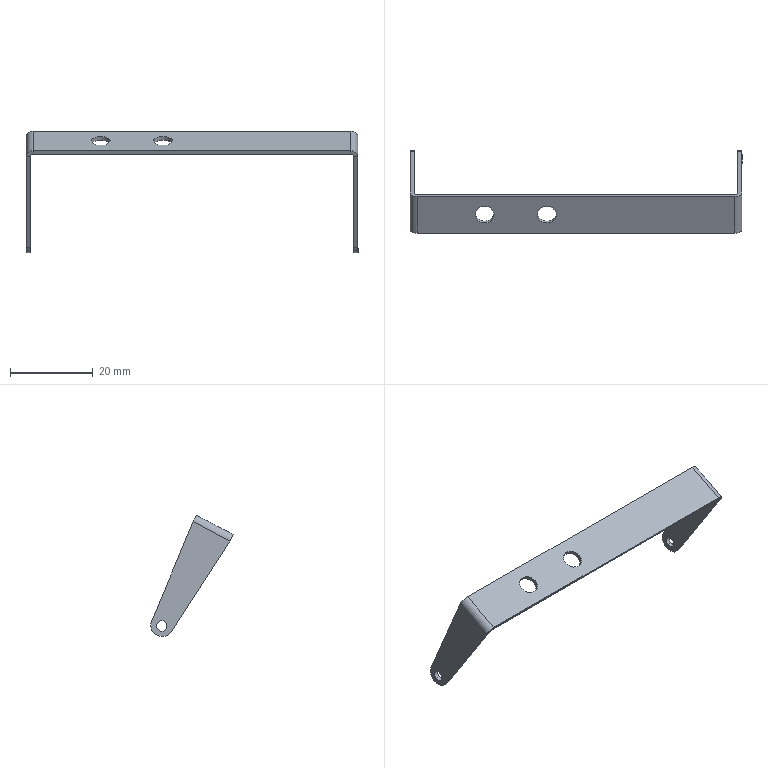Component | SolidWorks | ToolHolderAssembly-1_ToolHolder-1 | 1 solid | 34 faces | box 80 x 19.87 x 29.24 mm | volume 1182 mm3 | plane 18 | cylinder 16 | commonest cylinder face diameters 4.5 x4 2.5 x4 5.2 x4 3.473 x2 1.473 x2
STEP:
#1=COLOUR_RGB('',0.7922,0.8196,0.9333);
#2=FILL_AREA_STYLE_COLOUR('',#1);
#3=FILL_AREA_STYLE('',(#2));
#4=SURFACE_STYLE_FILL_AREA(#3);
#5=SURFACE_SIDE_STYLE('',(#4));
#6=SURFACE_STYLE_USAGE(.BOTH.,#5);
#7=PRESENTATION_STYLE_ASSIGNMENT((#6));
#8=CARTESIAN_POINT('',(-6.282,-0.2465,6.428));
#9=VERTEX_POINT('',#8);
#10=CARTESIAN_POINT('',(-6.105,-0.2465,6.428));
#11=VERTEX_POINT('',#10);
#12=CARTESIAN_POINT('',(-6.194,-0.2465,6.428));
#13=DIRECTION('',(-0.,-0.4648,0.8854));
#14=DIRECTION('',(1.,-0.,0.));
#15=AXIS2_PLACEMENT_3D('',#12,#13,#14);
#16=CIRCLE('',#15,0.08858);
#17=EDGE_CURVE('',#9,#11,#16,.T.);
#18=ORIENTED_EDGE('',*,*,#17,.F.);
#19=CARTESIAN_POINT('',(-6.282,-0.2648,6.463));
#20=VERTEX_POINT('',#19);
#21=CARTESIAN_POINT('',(-6.282,-0.2648,6.463));
#22=DIRECTION('',(-0.,-0.4648,0.8854));
#23=VECTOR('',#22,39.37);
#24=LINE('',#21,#23);
#25=EDGE_CURVE('',#9,#20,#24,.T.);
#26=ORIENTED_EDGE('',*,*,#25,.T.);
#27=CARTESIAN_POINT('',(-6.105,-0.2648,6.463));
#28=VERTEX_POINT('',#27);
#29=CARTESIAN_POINT('',(-6.194,-0.2648,6.463));
#30=DIRECTION('',(-0.,-0.4648,0.8854));
#31=DIRECTION('',(1.,-0.,0.));
#32=AXIS2_PLACEMENT_3D('',#29,#30,#31);
#33=CIRCLE('',#32,0.08858);
#34=EDGE_CURVE('',#20,#28,#33,.T.);
#35=ORIENTED_EDGE('',*,*,#34,.T.);
#36=CARTESIAN_POINT('',(-6.105,-0.2648,6.463));
#37=DIRECTION('',(-0.,-0.4648,0.8854));
#38=VECTOR('',#37,39.37);
#39=LINE('',#36,#38);
#40=EDGE_CURVE('',#11,#28,#39,.T.);
#41=ORIENTED_EDGE('',*,*,#40,.F.);
#42=EDGE_LOOP('',(#18,#26,#35,#41));
#43=FACE_OUTER_BOUND('',#42,.T.);
#44=CARTESIAN_POINT('',(-6.194,-0.2648,6.463));
#45=DIRECTION('',(-0.,-0.4648,0.8854));
#46=DIRECTION('',(1.,-0.,0.));
#47=AXIS2_PLACEMENT_3D('',#44,#45,#46);
#48=CYLINDRICAL_SURFACE('',#47,0.08858);
#49=ADVANCED_FACE('',(#43),#48,.F.);
#50=CARTESIAN_POINT('',(-6.873,-0.2465,6.428));
#51=VERTEX_POINT('',#50);
#52=CARTESIAN_POINT('',(-6.696,-0.2465,6.428));
#53=VERTEX_POINT('',#52);
#54=CARTESIAN_POINT('',(-6.784,-0.2465,6.428));
#55=DIRECTION('',(-0.,-0.4648,0.8854));
#56=DIRECTION('',(1.,-0.,0.));
#57=AXIS2_PLACEMENT_3D('',#54,#55,#56);
#58=CIRCLE('',#57,0.08858);
#59=EDGE_CURVE('',#51,#53,#58,.T.);
#60=ORIENTED_EDGE('',*,*,#59,.F.);
#61=CARTESIAN_POINT('',(-6.873,-0.2648,6.463));
#62=VERTEX_POINT('',#61);
#63=CARTESIAN_POINT('',(-6.873,-0.2648,6.463));
#64=DIRECTION('',(-0.,-0.4648,0.8854));
#65=VECTOR('',#64,39.37);
#66=LINE('',#63,#65);
#67=EDGE_CURVE('',#51,#62,#66,.T.);
#68=ORIENTED_EDGE('',*,*,#67,.T.);
#69=CARTESIAN_POINT('',(-6.696,-0.2648,6.463));
#70=VERTEX_POINT('',#69);
#71=CARTESIAN_POINT('',(-6.784,-0.2648,6.463));
#72=DIRECTION('',(-0.,-0.4648,0.8854));
#73=DIRECTION('',(1.,-0.,0.));
#74=AXIS2_PLACEMENT_3D('',#71,#72,#73);
#75=CIRCLE('',#74,0.08858);
#76=EDGE_CURVE('',#62,#70,#75,.T.);
#77=ORIENTED_EDGE('',*,*,#76,.T.);
#78=CARTESIAN_POINT('',(-6.696,-0.2648,6.463));
#79=DIRECTION('',(-0.,-0.4648,0.8854));
#80=VECTOR('',#79,39.37);
#81=LINE('',#78,#80);
#82=EDGE_CURVE('',#53,#70,#81,.T.);
#83=ORIENTED_EDGE('',*,*,#82,.F.);
#84=EDGE_LOOP('',(#60,#68,#77,#83));
#85=FACE_OUTER_BOUND('',#84,.T.);
#86=CARTESIAN_POINT('',(-6.784,-0.2648,6.463));
#87=DIRECTION('',(-0.,-0.4648,0.8854));
#88=DIRECTION('',(1.,-0.,0.));
#89=AXIS2_PLACEMENT_3D('',#86,#87,#88);
#90=CYLINDRICAL_SURFACE('',#89,0.08858);
#91=ADVANCED_FACE('',(#85),#90,.F.);
#92=CARTESIAN_POINT('',(-4.383,0.2613,5.461));
#93=VERTEX_POINT('',#92);
#94=CARTESIAN_POINT('',(-4.383,0.2155,5.548));
#95=VERTEX_POINT('',#94);
#96=CARTESIAN_POINT('',(-4.383,0.2384,5.504));
#97=DIRECTION('',(-1.,0.,-0.));
#98=DIRECTION('',(-0.,-0.4648,0.8854));
#99=AXIS2_PLACEMENT_3D('',#96,#97,#98);
#100=CIRCLE('',#99,0.04921);
#101=EDGE_CURVE('',#93,#95,#100,.T.);
#102=ORIENTED_EDGE('',*,*,#101,.T.);
#103=CARTESIAN_POINT('',(-4.343,0.2155,5.548));
#104=VERTEX_POINT('',#103);
#105=CARTESIAN_POINT('',(-7.493,0.2155,5.548));
#106=DIRECTION('',(1.,-0.,0.));
#107=VECTOR('',#106,39.37);
#108=LINE('',#105,#107);
#109=EDGE_CURVE('',#95,#104,#108,.T.);
#110=ORIENTED_EDGE('',*,*,#109,.T.);
#111=CARTESIAN_POINT('',(-4.343,0.2613,5.461));
#112=VERTEX_POINT('',#111);
#113=CARTESIAN_POINT('',(-4.343,0.2384,5.504));
#114=DIRECTION('',(1.,-0.,0.));
#115=DIRECTION('',(0.,0.4648,-0.8854));
#116=AXIS2_PLACEMENT_3D('',#113,#114,#115);
#117=CIRCLE('',#116,0.04921);
#118=EDGE_CURVE('',#104,#112,#117,.T.);
#119=ORIENTED_EDGE('',*,*,#118,.T.);
#120=CARTESIAN_POINT('',(-7.493,0.2613,5.461));
#121=DIRECTION('',(1.,-0.,0.));
#122=VECTOR('',#121,39.37);
#123=LINE('',#120,#122);
#124=EDGE_CURVE('',#93,#112,#123,.T.);
#125=ORIENTED_EDGE('',*,*,#124,.F.);
#126=EDGE_LOOP('',(#102,#110,#119,#125));
#127=FACE_OUTER_BOUND('',#126,.T.);
#128=CARTESIAN_POINT('',(-7.493,0.2384,5.504));
#129=DIRECTION('',(1.,-0.,0.));
#130=DIRECTION('',(0.,0.4648,-0.8854));
#131=AXIS2_PLACEMENT_3D('',#128,#129,#130);
#132=CYLINDRICAL_SURFACE('',#131,0.04921);
#133=ADVANCED_FACE('',(#127),#132,.F.);
#134=CARTESIAN_POINT('',(-7.493,0.2155,5.548));
#135=VERTEX_POINT('',#134);
#136=CARTESIAN_POINT('',(-7.493,0.2613,5.461));
#137=VERTEX_POINT('',#136);
#138=CARTESIAN_POINT('',(-7.493,0.2384,5.504));
#139=DIRECTION('',(1.,-0.,0.));
#140=DIRECTION('',(0.,0.4648,-0.8854));
#141=AXIS2_PLACEMENT_3D('',#138,#139,#140);
#142=CIRCLE('',#141,0.04921);
#143=EDGE_CURVE('',#135,#137,#142,.T.);
#144=ORIENTED_EDGE('',*,*,#143,.F.);
#145=CARTESIAN_POINT('',(-7.453,0.2155,5.548));
#146=VERTEX_POINT('',#145);
#147=CARTESIAN_POINT('',(-7.493,0.2155,5.548));
#148=DIRECTION('',(1.,-0.,0.));
#149=VECTOR('',#148,39.37);
#150=LINE('',#147,#149);
#151=EDGE_CURVE('',#135,#146,#150,.T.);
#152=ORIENTED_EDGE('',*,*,#151,.T.);
#153=CARTESIAN_POINT('',(-7.453,0.2613,5.461));
#154=VERTEX_POINT('',#153);
#155=CARTESIAN_POINT('',(-7.453,0.2384,5.504));
#156=DIRECTION('',(1.,-0.,0.));
#157=DIRECTION('',(0.,0.4648,-0.8854));
#158=AXIS2_PLACEMENT_3D('',#155,#156,#157);
#159=CIRCLE('',#158,0.04921);
#160=EDGE_CURVE('',#146,#154,#159,.T.);
#161=ORIENTED_EDGE('',*,*,#160,.T.);
#162=CARTESIAN_POINT('',(-7.493,0.2613,5.461));
#163=DIRECTION('',(1.,-0.,0.));
#164=VECTOR('',#163,39.37);
#165=LINE('',#162,#164);
#166=EDGE_CURVE('',#137,#154,#165,.T.);
#167=ORIENTED_EDGE('',*,*,#166,.F.);
#168=EDGE_LOOP('',(#144,#152,#161,#167));
#169=FACE_OUTER_BOUND('',#168,.T.);
#170=CARTESIAN_POINT('',(-7.493,0.2384,5.504));
#171=DIRECTION('',(1.,-0.,0.));
#172=DIRECTION('',(0.,0.4648,-0.8854));
#173=AXIS2_PLACEMENT_3D('',#170,#171,#172);
#174=CYLINDRICAL_SURFACE('',#173,0.04921);
#175=ADVANCED_FACE('',(#169),#174,.F.);
#176=CARTESIAN_POINT('',(-6.194,-0.2648,6.463));
#177=DIRECTION('',(-0.,-0.4648,0.8854));
#178=DIRECTION('',(1.,-0.,0.));
#179=AXIS2_PLACEMENT_3D('',#176,#177,#178);
#180=CIRCLE('',#179,0.08858);
#181=EDGE_CURVE('',#28,#20,#180,.T.);
#182=ORIENTED_EDGE('',*,*,#181,.F.);
#183=ORIENTED_EDGE('',*,*,#34,.F.);
#184=EDGE_LOOP('',(#182,#183));
#185=FACE_BOUND('',#184,.T.);
#186=CARTESIAN_POINT('',(-6.784,-0.2648,6.463));
#187=DIRECTION('',(-0.,-0.4648,0.8854));
#188=DIRECTION('',(1.,-0.,0.));
#189=AXIS2_PLACEMENT_3D('',#186,#187,#188);
#190=CIRCLE('',#189,0.08858);
#191=EDGE_CURVE('',#70,#62,#190,.T.);
#192=ORIENTED_EDGE('',*,*,#191,.F.);
#193=ORIENTED_EDGE('',*,*,#76,.F.);
#194=EDGE_LOOP('',(#192,#193));
#195=FACE_BOUND('',#194,.T.);
#196=CARTESIAN_POINT('',(-7.424,-0.09053,6.554));
#197=VERTEX_POINT('',#196);
#198=CARTESIAN_POINT('',(-4.412,-0.09053,6.554));
#199=VERTEX_POINT('',#198);
#200=CARTESIAN_POINT('',(-4.343,-0.09053,6.554));
#201=DIRECTION('',(1.,-0.,0.));
#202=VECTOR('',#201,39.37);
#203=LINE('',#200,#202);
#204=EDGE_CURVE('',#197,#199,#203,.T.);
#205=ORIENTED_EDGE('',*,*,#204,.F.);
#206=CARTESIAN_POINT('',(-7.424,-0.4391,6.371));
#207=VERTEX_POINT('',#206);
#208=CARTESIAN_POINT('',(-7.424,-0.09053,6.554));
#209=DIRECTION('',(0.,-0.8854,-0.4648));
#210=VECTOR('',#209,39.37);
#211=LINE('',#208,#210);
#212=EDGE_CURVE('',#197,#207,#211,.T.);
#213=ORIENTED_EDGE('',*,*,#212,.T.);
#214=CARTESIAN_POINT('',(-4.412,-0.4391,6.371));
#215=VERTEX_POINT('',#214);
#216=CARTESIAN_POINT('',(-4.343,-0.4391,6.371));
#217=DIRECTION('',(-1.,0.,-0.));
#218=VECTOR('',#217,39.37);
#219=LINE('',#216,#218);
#220=EDGE_CURVE('',#215,#207,#219,.T.);
#221=ORIENTED_EDGE('',*,*,#220,.F.);
#222=CARTESIAN_POINT('',(-4.412,-0.4391,6.371));
#223=DIRECTION('',(-0.,0.8854,0.4648));
#224=VECTOR('',#223,39.37);
#225=LINE('',#222,#224);
#226=EDGE_CURVE('',#215,#199,#225,.T.);
#227=ORIENTED_EDGE('',*,*,#226,.T.);
#228=EDGE_LOOP('',(#205,#213,#221,#227));
#229=FACE_OUTER_BOUND('',#228,.T.);
#230=CARTESIAN_POINT('',(-5.918,-0.2648,6.463));
#231=DIRECTION('',(-0.,-0.4648,0.8854));
#232=DIRECTION('',(1.,-0.,0.));
#233=AXIS2_PLACEMENT_3D('',#230,#231,#232);
#234=PLANE('',#233);
#235=ADVANCED_FACE('',(#185,#195,#229),#234,.T.);
#236=CARTESIAN_POINT('',(-6.194,-0.2465,6.428));
#237=DIRECTION('',(-0.,-0.4648,0.8854));
#238=DIRECTION('',(1.,-0.,0.));
#239=AXIS2_PLACEMENT_3D('',#236,#237,#238);
#240=CIRCLE('',#239,0.08858);
#241=EDGE_CURVE('',#11,#9,#240,.T.);
#242=ORIENTED_EDGE('',*,*,#241,.T.);
#243=ORIENTED_EDGE('',*,*,#17,.T.);
#244=EDGE_LOOP('',(#242,#243));
#245=FACE_BOUND('',#244,.T.);
#246=CARTESIAN_POINT('',(-6.784,-0.2465,6.428));
#247=DIRECTION('',(-0.,-0.4648,0.8854));
#248=DIRECTION('',(1.,-0.,0.));
#249=AXIS2_PLACEMENT_3D('',#246,#247,#248);
#250=CIRCLE('',#249,0.08858);
#251=EDGE_CURVE('',#53,#51,#250,.T.);
#252=ORIENTED_EDGE('',*,*,#251,.T.);
#253=ORIENTED_EDGE('',*,*,#59,.T.);
#254=EDGE_LOOP('',(#252,#253));
#255=FACE_BOUND('',#254,.T.);
#256=CARTESIAN_POINT('',(-7.424,-0.07223,6.52));
#257=VERTEX_POINT('',#256);
#258=CARTESIAN_POINT('',(-7.424,-0.4208,6.337));
#259=VERTEX_POINT('',#258);
#260=CARTESIAN_POINT('',(-7.424,-0.07223,6.52));
#261=DIRECTION('',(0.,-0.8854,-0.4648));
#262=VECTOR('',#261,39.37);
#263=LINE('',#260,#262);
#264=EDGE_CURVE('',#257,#259,#263,.T.);
#265=ORIENTED_EDGE('',*,*,#264,.F.);
#266=CARTESIAN_POINT('',(-4.412,-0.07223,6.52));
#267=VERTEX_POINT('',#266);
#268=CARTESIAN_POINT('',(-4.343,-0.07223,6.52));
#269=DIRECTION('',(1.,-0.,0.));
#270=VECTOR('',#269,39.37);
#271=LINE('',#268,#270);
#272=EDGE_CURVE('',#257,#267,#271,.T.);
#273=ORIENTED_EDGE('',*,*,#272,.T.);
#274=CARTESIAN_POINT('',(-4.412,-0.4208,6.337));
#275=VERTEX_POINT('',#274);
#276=CARTESIAN_POINT('',(-4.412,-0.4208,6.337));
#277=DIRECTION('',(-0.,0.8854,0.4648));
#278=VECTOR('',#277,39.37);
#279=LINE('',#276,#278);
#280=EDGE_CURVE('',#275,#267,#279,.T.);
#281=ORIENTED_EDGE('',*,*,#280,.F.);
#282=CARTESIAN_POINT('',(-4.343,-0.4208,6.337));
#283=DIRECTION('',(-1.,0.,-0.));
#284=VECTOR('',#283,39.37);
#285=LINE('',#282,#284);
#286=EDGE_CURVE('',#275,#259,#285,.T.);
#287=ORIENTED_EDGE('',*,*,#286,.T.);
#288=EDGE_LOOP('',(#265,#273,#281,#287));
#289=FACE_OUTER_BOUND('',#288,.T.);
#290=CARTESIAN_POINT('',(-5.918,-0.2465,6.428));
#291=DIRECTION('',(-0.,-0.4648,0.8854));
#292=DIRECTION('',(1.,-0.,0.));
#293=AXIS2_PLACEMENT_3D('',#290,#291,#292);
#294=PLANE('',#293);
#295=ADVANCED_FACE('',(#245,#255,#289),#294,.F.);
#296=ORIENTED_EDGE('',*,*,#272,.F.);
#297=CARTESIAN_POINT('',(-7.424,-0.07223,6.52));
#298=DIRECTION('',(-0.,-0.4648,0.8854));
#299=VECTOR('',#298,39.37);
#300=LINE('',#297,#299);
#301=EDGE_CURVE('',#257,#197,#300,.T.);
#302=ORIENTED_EDGE('',*,*,#301,.T.);
#303=ORIENTED_EDGE('',*,*,#204,.T.);
#304=CARTESIAN_POINT('',(-4.412,-0.07223,6.52));
#305=DIRECTION('',(-0.,-0.4648,0.8854));
#306=VECTOR('',#305,39.37);
#307=LINE('',#304,#306);
#308=EDGE_CURVE('',#267,#199,#307,.T.);
#309=ORIENTED_EDGE('',*,*,#308,.F.);
#310=EDGE_LOOP('',(#296,#302,#303,#309));
#311=FACE_OUTER_BOUND('',#310,.T.);
#312=CARTESIAN_POINT('',(-4.343,-0.09053,6.554));
#313=DIRECTION('',(-0.,0.8854,0.4648));
#314=DIRECTION('',(0.,0.4648,-0.8854));
#315=AXIS2_PLACEMENT_3D('',#312,#313,#314);
#316=PLANE('',#315);
#317=ADVANCED_FACE('',(#311),#316,.T.);
#318=CARTESIAN_POINT('',(-7.424,-0.4208,6.337));
#319=DIRECTION('',(-0.,-0.4648,0.8854));
#320=VECTOR('',#319,39.37);
#321=LINE('',#318,#320);
#322=EDGE_CURVE('',#259,#207,#321,.T.);
#323=ORIENTED_EDGE('',*,*,#322,.F.);
#324=ORIENTED_EDGE('',*,*,#286,.F.);
#325=CARTESIAN_POINT('',(-4.412,-0.4208,6.337));
#326=DIRECTION('',(-0.,-0.4648,0.8854));
#327=VECTOR('',#326,39.37);
#328=LINE('',#325,#327);
#329=EDGE_CURVE('',#275,#215,#328,.T.);
#330=ORIENTED_EDGE('',*,*,#329,.T.);
#331=ORIENTED_EDGE('',*,*,#220,.T.);
#332=EDGE_LOOP('',(#323,#324,#330,#331));
#333=FACE_OUTER_BOUND('',#332,.T.);
#334=CARTESIAN_POINT('',(-4.343,-0.4391,6.371));
#335=DIRECTION('',(0.,-0.8854,-0.4648));
#336=DIRECTION('',(-0.,-0.4648,0.8854));
#337=AXIS2_PLACEMENT_3D('',#334,#335,#336);
#338=PLANE('',#337);
#339=ADVANCED_FACE('',(#333),#338,.T.);
#340=CARTESIAN_POINT('',(-4.383,-0.05875,6.494));
#341=VERTEX_POINT('',#340);
#342=CARTESIAN_POINT('',(-4.343,-0.05875,6.494));
#343=VERTEX_POINT('',#342);
#344=CARTESIAN_POINT('',(-4.343,-0.05875,6.494));
#345=DIRECTION('',(1.,-0.,0.));
#346=VECTOR('',#345,39.37);
#347=LINE('',#344,#346);
#348=EDGE_CURVE('',#341,#343,#347,.T.);
#349=ORIENTED_EDGE('',*,*,#348,.F.);
#350=CARTESIAN_POINT('',(-4.412,-0.05875,6.494));
#351=DIRECTION('',(-0.,0.8854,0.4648));
#352=DIRECTION('',(-0.,-0.4648,0.8854));
#353=AXIS2_PLACEMENT_3D('',#350,#351,#352);
#354=CIRCLE('',#353,0.029);
#355=EDGE_CURVE('',#267,#341,#354,.T.);
#356=ORIENTED_EDGE('',*,*,#355,.F.);
#357=ORIENTED_EDGE('',*,*,#308,.T.);
#358=CARTESIAN_POINT('',(-4.412,-0.05875,6.494));
#359=DIRECTION('',(-0.,0.8854,0.4648));
#360=DIRECTION('',(-0.,-0.4648,0.8854));
#361=AXIS2_PLACEMENT_3D('',#358,#359,#360);
#362=CIRCLE('',#361,0.06837);
#363=EDGE_CURVE('',#199,#343,#362,.T.);
#364=ORIENTED_EDGE('',*,*,#363,.T.);
#365=EDGE_LOOP('',(#349,#356,#357,#364));
#366=FACE_OUTER_BOUND('',#365,.T.);
#367=CARTESIAN_POINT('',(-4.412,-0.05875,6.494));
#368=DIRECTION('',(-0.,0.8854,0.4648));
#369=DIRECTION('',(0.,0.4648,-0.8854));
#370=AXIS2_PLACEMENT_3D('',#367,#368,#369);
#371=PLANE('',#370);
#372=ADVANCED_FACE('',(#366),#371,.T.);
#373=CARTESIAN_POINT('',(-4.383,-0.4073,6.311));
#374=VERTEX_POINT('',#373);
#375=CARTESIAN_POINT('',(-4.412,-0.4073,6.311));
#376=DIRECTION('',(0.,-0.8854,-0.4648));
#377=DIRECTION('',(-0.,-0.4648,0.8854));
#378=AXIS2_PLACEMENT_3D('',#375,#376,#377);
#379=CIRCLE('',#378,0.029);
#380=EDGE_CURVE('',#374,#275,#379,.T.);
#381=ORIENTED_EDGE('',*,*,#380,.F.);
#382=CARTESIAN_POINT('',(-4.343,-0.4073,6.311));
#383=VERTEX_POINT('',#382);
#384=CARTESIAN_POINT('',(-4.383,-0.4073,6.311));
#385=DIRECTION('',(1.,-0.,0.));
#386=VECTOR('',#385,39.37);
#387=LINE('',#384,#386);
#388=EDGE_CURVE('',#374,#383,#387,.T.);
#389=ORIENTED_EDGE('',*,*,#388,.T.);
#390=CARTESIAN_POINT('',(-4.412,-0.4073,6.311));
#391=DIRECTION('',(0.,-0.8854,-0.4648));
#392=DIRECTION('',(-0.,-0.4648,0.8854));
#393=AXIS2_PLACEMENT_3D('',#390,#391,#392);
#394=CIRCLE('',#393,0.06837);
#395=EDGE_CURVE('',#383,#215,#394,.T.);
#396=ORIENTED_EDGE('',*,*,#395,.T.);
#397=ORIENTED_EDGE('',*,*,#329,.F.);
#398=EDGE_LOOP('',(#381,#389,#396,#397));
#399=FACE_OUTER_BOUND('',#398,.T.);
#400=CARTESIAN_POINT('',(-4.412,-0.4073,6.311));
#401=DIRECTION('',(-0.,0.8854,0.4648));
#402=DIRECTION('',(0.,0.4648,-0.8854));
#403=AXIS2_PLACEMENT_3D('',#400,#401,#402);
#404=PLANE('',#403);
#405=ADVANCED_FACE('',(#399),#404,.F.);
#406=ORIENTED_EDGE('',*,*,#226,.F.);
#407=ORIENTED_EDGE('',*,*,#395,.F.);
#408=CARTESIAN_POINT('',(-4.343,-0.05875,6.494));
#409=DIRECTION('',(-0.,0.8854,0.4648));
#410=VECTOR('',#409,39.37);
#411=LINE('',#408,#410);
#412=EDGE_CURVE('',#383,#343,#411,.T.);
#413=ORIENTED_EDGE('',*,*,#412,.T.);
#414=ORIENTED_EDGE('',*,*,#363,.F.);
#415=EDGE_LOOP('',(#406,#407,#413,#414));
#416=FACE_OUTER_BOUND('',#415,.T.);
#417=CARTESIAN_POINT('',(-4.412,-0.4073,6.311));
#418=DIRECTION('',(0.,-0.8854,-0.4648));
#419=DIRECTION('',(1.,-0.,0.));
#420=AXIS2_PLACEMENT_3D('',#417,#418,#419);
#421=CYLINDRICAL_SURFACE('',#420,0.06837);
#422=ADVANCED_FACE('',(#416),#421,.T.);
#423=ORIENTED_EDGE('',*,*,#280,.T.);
#424=ORIENTED_EDGE('',*,*,#355,.T.);
#425=CARTESIAN_POINT('',(-4.383,-0.05875,6.494));
#426=DIRECTION('',(0.,-0.8854,-0.4648));
#427=VECTOR('',#426,39.37);
#428=LINE('',#425,#427);
#429=EDGE_CURVE('',#341,#374,#428,.T.);
#430=ORIENTED_EDGE('',*,*,#429,.T.);
#431=ORIENTED_EDGE('',*,*,#380,.T.);
#432=EDGE_LOOP('',(#423,#424,#430,#431));
#433=FACE_OUTER_BOUND('',#432,.T.);
#434=CARTESIAN_POINT('',(-4.412,-0.4073,6.311));
#435=DIRECTION('',(0.,-0.8854,-0.4648));
#436=DIRECTION('',(1.,-0.,0.));
#437=AXIS2_PLACEMENT_3D('',#434,#435,#436);
#438=CYLINDRICAL_SURFACE('',#437,0.029);
#439=ADVANCED_FACE('',(#433),#438,.F.);
#440=CARTESIAN_POINT('',(-4.343,0.2384,5.504));
#441=DIRECTION('',(1.,-0.,0.));
#442=DIRECTION('',(0.,0.4648,-0.8854));
#443=AXIS2_PLACEMENT_3D('',#440,#441,#442);
#444=CIRCLE('',#443,0.04921);
#445=EDGE_CURVE('',#112,#104,#444,.T.);
#446=ORIENTED_EDGE('',*,*,#445,.F.);
#447=ORIENTED_EDGE('',*,*,#118,.F.);
#448=EDGE_LOOP('',(#446,#447));
#449=FACE_BOUND('',#448,.T.);
#450=CARTESIAN_POINT('',(-4.343,0.28,5.415));
#451=VERTEX_POINT('',#450);
#452=CARTESIAN_POINT('',(-4.343,0.2883,5.419));
#453=VERTEX_POINT('',#452);
#454=CARTESIAN_POINT('',(-4.343,0.2842,5.417));
#455=DIRECTION('',(-0.,0.8854,0.4648));
#456=VECTOR('',#455,39.37);
#457=LINE('',#454,#456);
#458=EDGE_CURVE('',#451,#453,#457,.T.);
#459=ORIENTED_EDGE('',*,*,#458,.T.);
#460=CARTESIAN_POINT('',(-4.343,0.3352,5.549));
#461=VERTEX_POINT('',#460);
#462=CARTESIAN_POINT('',(-4.343,0.2408,5.51));
#463=DIRECTION('',(1.,-0.,0.));
#464=DIRECTION('',(-0.,-0.4648,0.8854));
#465=AXIS2_PLACEMENT_3D('',#462,#463,#464);
#466=CIRCLE('',#465,0.1024);
#467=EDGE_CURVE('',#453,#461,#466,.T.);
#468=ORIENTED_EDGE('',*,*,#467,.T.);
#469=CARTESIAN_POINT('',(-4.343,-0.05875,6.494));
#470=DIRECTION('',(0.,0.385,-0.9229));
#471=VECTOR('',#470,39.37);
#472=LINE('',#469,#471);
#473=EDGE_CURVE('',#343,#461,#472,.T.);
#474=ORIENTED_EDGE('',*,*,#473,.F.);
#475=ORIENTED_EDGE('',*,*,#412,.F.);
#476=CARTESIAN_POINT('',(-4.343,0.1463,5.45));
#477=VERTEX_POINT('',#476);
#478=CARTESIAN_POINT('',(-4.343,-0.4073,6.311));
#479=DIRECTION('',(-0.,-0.541,0.841));
#480=VECTOR('',#479,39.37);
#481=LINE('',#478,#480);
#482=EDGE_CURVE('',#477,#383,#481,.T.);
#483=ORIENTED_EDGE('',*,*,#482,.F.);
#484=CARTESIAN_POINT('',(-4.343,0.2324,5.506));
#485=DIRECTION('',(1.,-0.,0.));
#486=DIRECTION('',(-0.,-0.4648,0.8854));
#487=AXIS2_PLACEMENT_3D('',#484,#485,#486);
#488=CIRCLE('',#487,0.1024);
#489=EDGE_CURVE('',#477,#451,#488,.T.);
#490=ORIENTED_EDGE('',*,*,#489,.T.);
#491=EDGE_LOOP('',(#459,#468,#474,#475,#483,#490));
#492=FACE_OUTER_BOUND('',#491,.T.);
#493=CARTESIAN_POINT('',(-4.343,-0.2465,6.428));
#494=DIRECTION('',(-1.,0.,-0.));
#495=DIRECTION('',(-0.,-0.4648,0.8854));
#496=AXIS2_PLACEMENT_3D('',#493,#494,#495);
#497=PLANE('',#496);
#498=ADVANCED_FACE('',(#449,#492),#497,.F.);
#499=ORIENTED_EDGE('',*,*,#101,.F.);
#500=CARTESIAN_POINT('',(-4.383,0.2384,5.504));
#501=DIRECTION('',(-1.,0.,-0.));
#502=DIRECTION('',(-0.,-0.4648,0.8854));
#503=AXIS2_PLACEMENT_3D('',#500,#501,#502);
#504=CIRCLE('',#503,0.04921);
#505=EDGE_CURVE('',#95,#93,#504,.T.);
#506=ORIENTED_EDGE('',*,*,#505,.F.);
#507=EDGE_LOOP('',(#499,#506));
#508=FACE_BOUND('',#507,.T.);
#509=CARTESIAN_POINT('',(-4.383,0.3352,5.549));
#510=VERTEX_POINT('',#509);
#511=CARTESIAN_POINT('',(-4.383,-0.0632,6.505));
#512=DIRECTION('',(-0.,-0.385,0.9229));
#513=VECTOR('',#512,39.37);
#514=LINE('',#511,#513);
#515=EDGE_CURVE('',#510,#341,#514,.T.);
#516=ORIENTED_EDGE('',*,*,#515,.F.);
#517=CARTESIAN_POINT('',(-4.383,0.2883,5.419));
#518=VERTEX_POINT('',#517);
#519=CARTESIAN_POINT('',(-4.383,0.2408,5.51));
#520=DIRECTION('',(-1.,0.,-0.));
#521=DIRECTION('',(-0.,-0.4648,0.8854));
#522=AXIS2_PLACEMENT_3D('',#519,#520,#521);
#523=CIRCLE('',#522,0.1024);
#524=EDGE_CURVE('',#510,#518,#523,.T.);
#525=ORIENTED_EDGE('',*,*,#524,.T.);
#526=CARTESIAN_POINT('',(-4.383,0.28,5.415));
#527=VERTEX_POINT('',#526);
#528=CARTESIAN_POINT('',(-4.383,0.4585,5.509));
#529=DIRECTION('',(-0.,0.8854,0.4648));
#530=VECTOR('',#529,39.37);
#531=LINE('',#528,#530);
#532=EDGE_CURVE('',#527,#518,#531,.T.);
#533=ORIENTED_EDGE('',*,*,#532,.F.);
#534=CARTESIAN_POINT('',(-4.383,0.1463,5.45));
#535=VERTEX_POINT('',#534);
#536=CARTESIAN_POINT('',(-4.383,0.2324,5.506));
#537=DIRECTION('',(-1.,0.,-0.));
#538=DIRECTION('',(-0.,-0.4648,0.8854));
#539=AXIS2_PLACEMENT_3D('',#536,#537,#538);
#540=CIRCLE('',#539,0.1024);
#541=EDGE_CURVE('',#527,#535,#540,.T.);
#542=ORIENTED_EDGE('',*,*,#541,.T.);
#543=CARTESIAN_POINT('',(-4.383,-0.4136,6.321));
#544=DIRECTION('',(0.,0.541,-0.841));
#545=VECTOR('',#544,39.37);
#546=LINE('',#543,#545);
#547=EDGE_CURVE('',#374,#535,#546,.T.);
#548=ORIENTED_EDGE('',*,*,#547,.F.);
#549=ORIENTED_EDGE('',*,*,#429,.F.);
#550=EDGE_LOOP('',(#516,#525,#533,#542,#548,#549));
#551=FACE_OUTER_BOUND('',#550,.T.);
#552=CARTESIAN_POINT('',(-4.383,-0.2465,6.428));
#553=DIRECTION('',(-1.,0.,-0.));
#554=DIRECTION('',(-0.,-0.4648,0.8854));
#555=AXIS2_PLACEMENT_3D('',#552,#553,#554);
#556=PLANE('',#555);
#557=ADVANCED_FACE('',(#508,#551),#556,.T.);
#558=ORIENTED_EDGE('',*,*,#532,.T.);
#559=CARTESIAN_POINT('',(-4.343,0.2883,5.419));
#560=DIRECTION('',(1.,-0.,0.));
#561=VECTOR('',#560,39.37);
#562=LINE('',#559,#561);
#563=EDGE_CURVE('',#518,#453,#562,.T.);
#564=ORIENTED_EDGE('',*,*,#563,.T.);
#565=ORIENTED_EDGE('',*,*,#458,.F.);
#566=CARTESIAN_POINT('',(-4.343,0.28,5.415));
#567=DIRECTION('',(-1.,0.,-0.));
#568=VECTOR('',#567,39.37);
#569=LINE('',#566,#568);
#570=EDGE_CURVE('',#451,#527,#569,.T.);
#571=ORIENTED_EDGE('',*,*,#570,.T.);
#572=EDGE_LOOP('',(#558,#564,#565,#571));
#573=FACE_OUTER_BOUND('',#572,.T.);
#574=CARTESIAN_POINT('',(-4.343,0.4585,5.509));
#575=DIRECTION('',(-0.,-0.4648,0.8854));
#576=DIRECTION('',(1.,-0.,0.));
#577=AXIS2_PLACEMENT_3D('',#574,#575,#576);
#578=PLANE('',#577);
#579=ADVANCED_FACE('',(#573),#578,.F.);
#580=CARTESIAN_POINT('',(-7.453,-0.4073,6.311));
#581=VERTEX_POINT('',#580);
#582=CARTESIAN_POINT('',(-7.493,-0.4073,6.311));
#583=VERTEX_POINT('',#582);
#584=CARTESIAN_POINT('',(-7.493,-0.4073,6.311));
#585=DIRECTION('',(-1.,0.,-0.));
#586=VECTOR('',#585,39.37);
#587=LINE('',#584,#586);
#588=EDGE_CURVE('',#581,#583,#587,.T.);
#589=ORIENTED_EDGE('',*,*,#588,.F.);
#590=CARTESIAN_POINT('',(-7.424,-0.4073,6.311));
#591=DIRECTION('',(0.,-0.8854,-0.4648));
#592=DIRECTION('',(0.,0.4648,-0.8854));
#593=AXIS2_PLACEMENT_3D('',#590,#591,#592);
#594=CIRCLE('',#593,0.029);
#595=EDGE_CURVE('',#259,#581,#594,.T.);
#596=ORIENTED_EDGE('',*,*,#595,.F.);
#597=ORIENTED_EDGE('',*,*,#322,.T.);
#598=CARTESIAN_POINT('',(-7.424,-0.4073,6.311));
#599=DIRECTION('',(0.,-0.8854,-0.4648));
#600=DIRECTION('',(0.,0.4648,-0.8854));
#601=AXIS2_PLACEMENT_3D('',#598,#599,#600);
#602=CIRCLE('',#601,0.06837);
#603=EDGE_CURVE('',#207,#583,#602,.T.);
#604=ORIENTED_EDGE('',*,*,#603,.T.);
#605=EDGE_LOOP('',(#589,#596,#597,#604));
#606=FACE_OUTER_BOUND('',#605,.T.);
#607=CARTESIAN_POINT('',(-7.424,-0.4073,6.311));
#608=DIRECTION('',(0.,-0.8854,-0.4648));
#609=DIRECTION('',(-0.,-0.4648,0.8854));
#610=AXIS2_PLACEMENT_3D('',#607,#608,#609);
#611=PLANE('',#610);
#612=ADVANCED_FACE('',(#606),#611,.T.);
#613=CARTESIAN_POINT('',(-7.453,-0.05875,6.494));
#614=VERTEX_POINT('',#613);
#615=CARTESIAN_POINT('',(-7.424,-0.05875,6.494));
#616=DIRECTION('',(-0.,0.8854,0.4648));
#617=DIRECTION('',(0.,0.4648,-0.8854));
#618=AXIS2_PLACEMENT_3D('',#615,#616,#617);
#619=CIRCLE('',#618,0.029);
#620=EDGE_CURVE('',#614,#257,#619,.T.);
#621=ORIENTED_EDGE('',*,*,#620,.F.);
#622=CARTESIAN_POINT('',(-7.493,-0.05875,6.494));
#623=VERTEX_POINT('',#622);
#624=CARTESIAN_POINT('',(-7.453,-0.05875,6.494));
#625=DIRECTION('',(-1.,0.,-0.));
#626=VECTOR('',#625,39.37);
#627=LINE('',#624,#626);
#628=EDGE_CURVE('',#614,#623,#627,.T.);
#629=ORIENTED_EDGE('',*,*,#628,.T.);
#630=CARTESIAN_POINT('',(-7.424,-0.05875,6.494));
#631=DIRECTION('',(-0.,0.8854,0.4648));
#632=DIRECTION('',(0.,0.4648,-0.8854));
#633=AXIS2_PLACEMENT_3D('',#630,#631,#632);
#634=CIRCLE('',#633,0.06837);
#635=EDGE_CURVE('',#623,#197,#634,.T.);
#636=ORIENTED_EDGE('',*,*,#635,.T.);
#637=ORIENTED_EDGE('',*,*,#301,.F.);
#638=EDGE_LOOP('',(#621,#629,#636,#637));
#639=FACE_OUTER_BOUND('',#638,.T.);
#640=CARTESIAN_POINT('',(-7.424,-0.05875,6.494));
#641=DIRECTION('',(0.,-0.8854,-0.4648));
#642=DIRECTION('',(-0.,-0.4648,0.8854));
#643=AXIS2_PLACEMENT_3D('',#640,#641,#642);
#644=PLANE('',#643);
#645=ADVANCED_FACE('',(#639),#644,.F.);
#646=ORIENTED_EDGE('',*,*,#212,.F.);
#647=ORIENTED_EDGE('',*,*,#635,.F.);
#648=CARTESIAN_POINT('',(-7.493,-0.4073,6.311));
#649=DIRECTION('',(0.,-0.8854,-0.4648));
#650=VECTOR('',#649,39.37);
#651=LINE('',#648,#650);
#652=EDGE_CURVE('',#623,#583,#651,.T.);
#653=ORIENTED_EDGE('',*,*,#652,.T.);
#654=ORIENTED_EDGE('',*,*,#603,.F.);
#655=EDGE_LOOP('',(#646,#647,#653,#654));
#656=FACE_OUTER_BOUND('',#655,.T.);
#657=CARTESIAN_POINT('',(-7.424,-0.05875,6.494));
#658=DIRECTION('',(-0.,0.8854,0.4648));
#659=DIRECTION('',(-1.,0.,-0.));
#660=AXIS2_PLACEMENT_3D('',#657,#658,#659);
#661=CYLINDRICAL_SURFACE('',#660,0.06837);
#662=ADVANCED_FACE('',(#656),#661,.T.);
#663=ORIENTED_EDGE('',*,*,#264,.T.);
#664=ORIENTED_EDGE('',*,*,#595,.T.);
#665=CARTESIAN_POINT('',(-7.453,-0.4073,6.311));
#666=DIRECTION('',(-0.,0.8854,0.4648));
#667=VECTOR('',#666,39.37);
#668=LINE('',#665,#667);
#669=EDGE_CURVE('',#581,#614,#668,.T.);
#670=ORIENTED_EDGE('',*,*,#669,.T.);
#671=ORIENTED_EDGE('',*,*,#620,.T.);
#672=EDGE_LOOP('',(#663,#664,#670,#671));
#673=FACE_OUTER_BOUND('',#672,.T.);
#674=CARTESIAN_POINT('',(-7.424,-0.05875,6.494));
#675=DIRECTION('',(-0.,0.8854,0.4648));
#676=DIRECTION('',(-1.,0.,-0.));
#677=AXIS2_PLACEMENT_3D('',#674,#675,#676);
#678=CYLINDRICAL_SURFACE('',#677,0.029);
#679=ADVANCED_FACE('',(#673),#678,.F.);
#680=CARTESIAN_POINT('',(-7.493,0.2384,5.504));
#681=DIRECTION('',(1.,-0.,0.));
#682=DIRECTION('',(0.,0.4648,-0.8854));
#683=AXIS2_PLACEMENT_3D('',#680,#681,#682);
#684=CIRCLE('',#683,0.04921);
#685=EDGE_CURVE('',#137,#135,#684,.T.);
#686=ORIENTED_EDGE('',*,*,#685,.T.);
#687=ORIENTED_EDGE('',*,*,#143,.T.);
#688=EDGE_LOOP('',(#686,#687));
#689=FACE_BOUND('',#688,.T.);
#690=CARTESIAN_POINT('',(-7.493,0.3352,5.549));
#691=VERTEX_POINT('',#690);
#692=CARTESIAN_POINT('',(-7.493,-0.05875,6.494));
#693=DIRECTION('',(0.,0.385,-0.9229));
#694=VECTOR('',#693,39.37);
#695=LINE('',#692,#694);
#696=EDGE_CURVE('',#623,#691,#695,.T.);
#697=ORIENTED_EDGE('',*,*,#696,.T.);
#698=CARTESIAN_POINT('',(-7.493,0.2883,5.419));
#699=VERTEX_POINT('',#698);
#700=CARTESIAN_POINT('',(-7.493,0.2408,5.51));
#701=DIRECTION('',(-1.,0.,-0.));
#702=DIRECTION('',(0.,0.4648,-0.8854));
#703=AXIS2_PLACEMENT_3D('',#700,#701,#702);
#704=CIRCLE('',#703,0.1024);
#705=EDGE_CURVE('',#691,#699,#704,.T.);
#706=ORIENTED_EDGE('',*,*,#705,.T.);
#707=CARTESIAN_POINT('',(-7.493,0.28,5.415));
#708=VERTEX_POINT('',#707);
#709=CARTESIAN_POINT('',(-7.493,0.2842,5.417));
#710=DIRECTION('',(0.,-0.8854,-0.4648));
#711=VECTOR('',#710,39.37);
#712=LINE('',#709,#711);
#713=EDGE_CURVE('',#699,#708,#712,.T.);
#714=ORIENTED_EDGE('',*,*,#713,.T.);
#715=CARTESIAN_POINT('',(-7.493,0.1463,5.45));
#716=VERTEX_POINT('',#715);
#717=CARTESIAN_POINT('',(-7.493,0.2324,5.506));
#718=DIRECTION('',(-1.,0.,-0.));
#719=DIRECTION('',(0.,0.4648,-0.8854));
#720=AXIS2_PLACEMENT_3D('',#717,#718,#719);
#721=CIRCLE('',#720,0.1024);
#722=EDGE_CURVE('',#708,#716,#721,.T.);
#723=ORIENTED_EDGE('',*,*,#722,.T.);
#724=CARTESIAN_POINT('',(-7.493,-0.4073,6.311));
#725=DIRECTION('',(-0.,-0.541,0.841));
#726=VECTOR('',#725,39.37);
#727=LINE('',#724,#726);
#728=EDGE_CURVE('',#716,#583,#727,.T.);
#729=ORIENTED_EDGE('',*,*,#728,.T.);
#730=ORIENTED_EDGE('',*,*,#652,.F.);
#731=EDGE_LOOP('',(#697,#706,#714,#723,#729,#730));
#732=FACE_OUTER_BOUND('',#731,.T.);
#733=CARTESIAN_POINT('',(-7.493,-0.2465,6.428));
#734=DIRECTION('',(1.,-0.,0.));
#735=DIRECTION('',(0.,0.4648,-0.8854));
#736=AXIS2_PLACEMENT_3D('',#733,#734,#735);
#737=PLANE('',#736);
#738=ADVANCED_FACE('',(#689,#732),#737,.F.);
#739=CARTESIAN_POINT('',(-7.453,0.2384,5.504));
#740=DIRECTION('',(1.,-0.,0.));
#741=DIRECTION('',(0.,0.4648,-0.8854));
#742=AXIS2_PLACEMENT_3D('',#739,#740,#741);
#743=CIRCLE('',#742,0.04921);
#744=EDGE_CURVE('',#154,#146,#743,.T.);
#745=ORIENTED_EDGE('',*,*,#744,.F.);
#746=ORIENTED_EDGE('',*,*,#160,.F.);
#747=EDGE_LOOP('',(#745,#746));
#748=FACE_BOUND('',#747,.T.);
#749=CARTESIAN_POINT('',(-7.453,0.2883,5.419));
#750=VERTEX_POINT('',#749);
#751=CARTESIAN_POINT('',(-7.453,0.28,5.415));
#752=VERTEX_POINT('',#751);
#753=CARTESIAN_POINT('',(-7.453,0.1099,5.326));
#754=DIRECTION('',(0.,-0.8854,-0.4648));
#755=VECTOR('',#754,39.37);
#756=LINE('',#753,#755);
#757=EDGE_CURVE('',#750,#752,#756,.T.);
#758=ORIENTED_EDGE('',*,*,#757,.F.);
#759=CARTESIAN_POINT('',(-7.453,0.3352,5.549));
#760=VERTEX_POINT('',#759);
#761=CARTESIAN_POINT('',(-7.453,0.2408,5.51));
#762=DIRECTION('',(1.,-0.,0.));
#763=DIRECTION('',(0.,0.4648,-0.8854));
#764=AXIS2_PLACEMENT_3D('',#761,#762,#763);
#765=CIRCLE('',#764,0.1024);
#766=EDGE_CURVE('',#750,#760,#765,.T.);
#767=ORIENTED_EDGE('',*,*,#766,.T.);
#768=CARTESIAN_POINT('',(-7.453,-0.0632,6.505));
#769=DIRECTION('',(0.,0.385,-0.9229));
#770=VECTOR('',#769,39.37);
#771=LINE('',#768,#770);
#772=EDGE_CURVE('',#614,#760,#771,.T.);
#773=ORIENTED_EDGE('',*,*,#772,.F.);
#774=ORIENTED_EDGE('',*,*,#669,.F.);
#775=CARTESIAN_POINT('',(-7.453,0.1463,5.45));
#776=VERTEX_POINT('',#775);
#777=CARTESIAN_POINT('',(-7.453,-0.4136,6.321));
#778=DIRECTION('',(-0.,-0.541,0.841));
#779=VECTOR('',#778,39.37);
#780=LINE('',#777,#779);
#781=EDGE_CURVE('',#776,#581,#780,.T.);
#782=ORIENTED_EDGE('',*,*,#781,.F.);
#783=CARTESIAN_POINT('',(-7.453,0.2324,5.506));
#784=DIRECTION('',(1.,-0.,0.));
#785=DIRECTION('',(0.,0.4648,-0.8854));
#786=AXIS2_PLACEMENT_3D('',#783,#784,#785);
#787=CIRCLE('',#786,0.1024);
#788=EDGE_CURVE('',#776,#752,#787,.T.);
#789=ORIENTED_EDGE('',*,*,#788,.T.);
#790=EDGE_LOOP('',(#758,#767,#773,#774,#782,#789));
#791=FACE_OUTER_BOUND('',#790,.T.);
#792=CARTESIAN_POINT('',(-7.453,-0.2465,6.428));
#793=DIRECTION('',(1.,-0.,0.));
#794=DIRECTION('',(0.,0.4648,-0.8854));
#795=AXIS2_PLACEMENT_3D('',#792,#793,#794);
#796=PLANE('',#795);
#797=ADVANCED_FACE('',(#748,#791),#796,.T.);
#798=ORIENTED_EDGE('',*,*,#713,.F.);
#799=CARTESIAN_POINT('',(-7.493,0.2883,5.419));
#800=DIRECTION('',(1.,-0.,0.));
#801=VECTOR('',#800,39.37);
#802=LINE('',#799,#801);
#803=EDGE_CURVE('',#699,#750,#802,.T.);
#804=ORIENTED_EDGE('',*,*,#803,.T.);
#805=ORIENTED_EDGE('',*,*,#757,.T.);
#806=CARTESIAN_POINT('',(-7.493,0.28,5.415));
#807=DIRECTION('',(-1.,0.,-0.));
#808=VECTOR('',#807,39.37);
#809=LINE('',#806,#808);
#810=EDGE_CURVE('',#752,#708,#809,.T.);
#811=ORIENTED_EDGE('',*,*,#810,.T.);
#812=EDGE_LOOP('',(#798,#804,#805,#811));
#813=FACE_OUTER_BOUND('',#812,.T.);
#814=CARTESIAN_POINT('',(-7.493,0.1099,5.326));
#815=DIRECTION('',(-0.,-0.4648,0.8854));
#816=DIRECTION('',(1.,-0.,0.));
#817=AXIS2_PLACEMENT_3D('',#814,#815,#816);
#818=PLANE('',#817);
#819=ADVANCED_FACE('',(#813),#818,.F.);
#820=ORIENTED_EDGE('',*,*,#728,.F.);
#821=CARTESIAN_POINT('',(-7.493,0.1463,5.45));
#822=DIRECTION('',(1.,-0.,0.));
#823=VECTOR('',#822,39.37);
#824=LINE('',#821,#823);
#825=EDGE_CURVE('',#716,#776,#824,.T.);
#826=ORIENTED_EDGE('',*,*,#825,.T.);
#827=ORIENTED_EDGE('',*,*,#781,.T.);
#828=ORIENTED_EDGE('',*,*,#588,.T.);
#829=EDGE_LOOP('',(#820,#826,#827,#828));
#830=FACE_OUTER_BOUND('',#829,.T.);
#831=CARTESIAN_POINT('',(-7.493,-0.4073,6.311));
#832=DIRECTION('',(-0.,0.841,0.541));
#833=DIRECTION('',(0.,0.541,-0.841));
#834=AXIS2_PLACEMENT_3D('',#831,#832,#833);
#835=PLANE('',#834);
#836=ADVANCED_FACE('',(#830),#835,.F.);
#837=ORIENTED_EDGE('',*,*,#772,.T.);
#838=CARTESIAN_POINT('',(-7.493,0.3352,5.549));
#839=DIRECTION('',(-1.,0.,-0.));
#840=VECTOR('',#839,39.37);
#841=LINE('',#838,#840);
#842=EDGE_CURVE('',#760,#691,#841,.T.);
#843=ORIENTED_EDGE('',*,*,#842,.T.);
#844=ORIENTED_EDGE('',*,*,#696,.F.);
#845=ORIENTED_EDGE('',*,*,#628,.F.);
#846=EDGE_LOOP('',(#837,#843,#844,#845));
#847=FACE_OUTER_BOUND('',#846,.T.);
#848=CARTESIAN_POINT('',(-7.493,-0.05875,6.494));
#849=DIRECTION('',(0.,-0.9229,-0.385));
#850=DIRECTION('',(-0.,-0.385,0.9229));
#851=AXIS2_PLACEMENT_3D('',#848,#849,#850);
#852=PLANE('',#851);
#853=ADVANCED_FACE('',(#847),#852,.F.);
#854=ORIENTED_EDGE('',*,*,#547,.T.);
#855=CARTESIAN_POINT('',(-7.493,0.1463,5.45));
#856=DIRECTION('',(1.,-0.,0.));
#857=VECTOR('',#856,39.37);
#858=LINE('',#855,#857);
#859=EDGE_CURVE('',#535,#477,#858,.T.);
#860=ORIENTED_EDGE('',*,*,#859,.T.);
#861=ORIENTED_EDGE('',*,*,#482,.T.);
#862=ORIENTED_EDGE('',*,*,#388,.F.);
#863=EDGE_LOOP('',(#854,#860,#861,#862));
#864=FACE_OUTER_BOUND('',#863,.T.);
#865=CARTESIAN_POINT('',(-7.493,-0.4073,6.311));
#866=DIRECTION('',(-0.,0.841,0.541));
#867=DIRECTION('',(0.,0.541,-0.841));
#868=AXIS2_PLACEMENT_3D('',#865,#866,#867);
#869=PLANE('',#868);
#870=ADVANCED_FACE('',(#864),#869,.F.);
#871=ORIENTED_EDGE('',*,*,#473,.T.);
#872=CARTESIAN_POINT('',(-7.493,0.3352,5.549));
#873=DIRECTION('',(-1.,0.,-0.));
#874=VECTOR('',#873,39.37);
#875=LINE('',#872,#874);
#876=EDGE_CURVE('',#461,#510,#875,.T.);
#877=ORIENTED_EDGE('',*,*,#876,.T.);
#878=ORIENTED_EDGE('',*,*,#515,.T.);
#879=ORIENTED_EDGE('',*,*,#348,.T.);
#880=EDGE_LOOP('',(#871,#877,#878,#879));
#881=FACE_OUTER_BOUND('',#880,.T.);
#882=CARTESIAN_POINT('',(-7.493,-0.05875,6.494));
#883=DIRECTION('',(0.,-0.9229,-0.385));
#884=DIRECTION('',(-0.,-0.385,0.9229));
#885=AXIS2_PLACEMENT_3D('',#882,#883,#884);
#886=PLANE('',#885);
#887=ADVANCED_FACE('',(#881),#886,.F.);
#888=ORIENTED_EDGE('',*,*,#705,.F.);
#889=ORIENTED_EDGE('',*,*,#842,.F.);
#890=ORIENTED_EDGE('',*,*,#766,.F.);
#891=ORIENTED_EDGE('',*,*,#803,.F.);
#892=EDGE_LOOP('',(#888,#889,#890,#891));
#893=FACE_OUTER_BOUND('',#892,.T.);
#894=CARTESIAN_POINT('',(-7.493,0.2408,5.51));
#895=DIRECTION('',(1.,-0.,0.));
#896=DIRECTION('',(0.,0.4648,-0.8854));
#897=AXIS2_PLACEMENT_3D('',#894,#895,#896);
#898=CYLINDRICAL_SURFACE('',#897,0.1024);
#899=ADVANCED_FACE('',(#893),#898,.T.);
#900=ORIENTED_EDGE('',*,*,#722,.F.);
#901=ORIENTED_EDGE('',*,*,#810,.F.);
#902=ORIENTED_EDGE('',*,*,#788,.F.);
#903=ORIENTED_EDGE('',*,*,#825,.F.);
#904=EDGE_LOOP('',(#900,#901,#902,#903));
#905=FACE_OUTER_BOUND('',#904,.T.);
#906=CARTESIAN_POINT('',(-7.493,0.2324,5.506));
#907=DIRECTION('',(1.,-0.,0.));
#908=DIRECTION('',(0.,0.4648,-0.8854));
#909=AXIS2_PLACEMENT_3D('',#906,#907,#908);
#910=CYLINDRICAL_SURFACE('',#909,0.1024);
#911=ADVANCED_FACE('',(#905),#910,.T.);
#912=ORIENTED_EDGE('',*,*,#524,.F.);
#913=ORIENTED_EDGE('',*,*,#876,.F.);
#914=ORIENTED_EDGE('',*,*,#467,.F.);
#915=ORIENTED_EDGE('',*,*,#563,.F.);
#916=EDGE_LOOP('',(#912,#913,#914,#915));
#917=FACE_OUTER_BOUND('',#916,.T.);
#918=CARTESIAN_POINT('',(-4.343,0.2408,5.51));
#919=DIRECTION('',(1.,-0.,0.));
#920=DIRECTION('',(0.,0.4648,-0.8854));
#921=AXIS2_PLACEMENT_3D('',#918,#919,#920);
#922=CYLINDRICAL_SURFACE('',#921,0.1024);
#923=ADVANCED_FACE('',(#917),#922,.T.);
#924=ORIENTED_EDGE('',*,*,#541,.F.);
#925=ORIENTED_EDGE('',*,*,#570,.F.);
#926=ORIENTED_EDGE('',*,*,#489,.F.);
#927=ORIENTED_EDGE('',*,*,#859,.F.);
#928=EDGE_LOOP('',(#924,#925,#926,#927));
#929=FACE_OUTER_BOUND('',#928,.T.);
#930=CARTESIAN_POINT('',(-7.493,0.2324,5.506));
#931=DIRECTION('',(1.,-0.,0.));
#932=DIRECTION('',(0.,0.4648,-0.8854));
#933=AXIS2_PLACEMENT_3D('',#930,#931,#932);
#934=CYLINDRICAL_SURFACE('',#933,0.1024);
#935=ADVANCED_FACE('',(#929),#934,.T.);
#936=ORIENTED_EDGE('',*,*,#151,.F.);
#937=ORIENTED_EDGE('',*,*,#685,.F.);
#938=ORIENTED_EDGE('',*,*,#166,.T.);
#939=ORIENTED_EDGE('',*,*,#744,.T.);
#940=EDGE_LOOP('',(#936,#937,#938,#939));
#941=FACE_OUTER_BOUND('',#940,.T.);
#942=CARTESIAN_POINT('',(-7.493,0.2384,5.504));
#943=DIRECTION('',(1.,-0.,0.));
#944=DIRECTION('',(0.,0.4648,-0.8854));
#945=AXIS2_PLACEMENT_3D('',#942,#943,#944);
#946=CYLINDRICAL_SURFACE('',#945,0.04921);
#947=ADVANCED_FACE('',(#941),#946,.F.);
#948=ORIENTED_EDGE('',*,*,#109,.F.);
#949=ORIENTED_EDGE('',*,*,#505,.T.);
#950=ORIENTED_EDGE('',*,*,#124,.T.);
#951=ORIENTED_EDGE('',*,*,#445,.T.);
#952=EDGE_LOOP('',(#948,#949,#950,#951));
#953=FACE_OUTER_BOUND('',#952,.T.);
#954=CARTESIAN_POINT('',(-7.493,0.2384,5.504));
#955=DIRECTION('',(1.,-0.,0.));
#956=DIRECTION('',(0.,0.4648,-0.8854));
#957=AXIS2_PLACEMENT_3D('',#954,#955,#956);
#958=CYLINDRICAL_SURFACE('',#957,0.04921);
#959=ADVANCED_FACE('',(#953),#958,.F.);
#960=ORIENTED_EDGE('',*,*,#67,.F.);
#961=ORIENTED_EDGE('',*,*,#251,.F.);
#962=ORIENTED_EDGE('',*,*,#82,.T.);
#963=ORIENTED_EDGE('',*,*,#191,.T.);
#964=EDGE_LOOP('',(#960,#961,#962,#963));
#965=FACE_OUTER_BOUND('',#964,.T.);
#966=CARTESIAN_POINT('',(-6.784,-0.2648,6.463));
#967=DIRECTION('',(-0.,-0.4648,0.8854));
#968=DIRECTION('',(1.,-0.,0.));
#969=AXIS2_PLACEMENT_3D('',#966,#967,#968);
#970=CYLINDRICAL_SURFACE('',#969,0.08858);
#971=ADVANCED_FACE('',(#965),#970,.F.);
#972=ORIENTED_EDGE('',*,*,#25,.F.);
#973=ORIENTED_EDGE('',*,*,#241,.F.);
#974=ORIENTED_EDGE('',*,*,#40,.T.);
#975=ORIENTED_EDGE('',*,*,#181,.T.);
#976=EDGE_LOOP('',(#972,#973,#974,#975));
#977=FACE_OUTER_BOUND('',#976,.T.);
#978=CARTESIAN_POINT('',(-6.194,-0.2648,6.463));
#979=DIRECTION('',(-0.,-0.4648,0.8854));
#980=DIRECTION('',(1.,-0.,0.));
#981=AXIS2_PLACEMENT_3D('',#978,#979,#980);
#982=CYLINDRICAL_SURFACE('',#981,0.08858);
#983=ADVANCED_FACE('',(#977),#982,.F.);
#984=CLOSED_SHELL('',(#49,#91,#133,#175,#235,#295,#317,#339,#372,#405,#422,#439,#498,#557,#579,#612,#645,#662,#679,#738,#797,#819,#836,#853,#870,#887,#899,#911,#923,#935,#947,#959,#971,#983));
#985=MANIFOLD_SOLID_BREP('',#984);
#986=STYLED_ITEM('',(#7),#985);
#987=PRESENTATION_LAYER_ASSIGNMENT('','',(#986));
#988=(LENGTH_UNIT()NAMED_UNIT(*)SI_UNIT($,.METRE.));
#989=LENGTH_MEASURE_WITH_UNIT(LENGTH_MEASURE(0.0254),#988);
#990=DIMENSIONAL_EXPONENTS(1.,0.,0.,0.,0.,0.,0.);
#991=(CONVERSION_BASED_UNIT('',#989)LENGTH_UNIT()NAMED_UNIT(#990));
#992=UNCERTAINTY_MEASURE_WITH_UNIT(LENGTH_MEASURE(0.00001),#991,'','');
#993=(NAMED_UNIT(*)PLANE_ANGLE_UNIT()SI_UNIT($,.RADIAN.));
#994=(NAMED_UNIT(*)SI_UNIT($,.STERADIAN.)SOLID_ANGLE_UNIT());
#995=(GEOMETRIC_REPRESENTATION_CONTEXT(3)GLOBAL_UNCERTAINTY_ASSIGNED_CONTEXT((#992))GLOBAL_UNIT_ASSIGNED_CONTEXT((#991,#993,#994))REPRESENTATION_CONTEXT('',''));
#996=MECHANICAL_DESIGN_GEOMETRIC_PRESENTATION_REPRESENTATION('',(#986),#995);
#997=CARTESIAN_POINT('',(0.,0.,0.));
#998=DIRECTION('',(0.,0.,1.));
#999=DIRECTION('',(1.,0.,0.));
#1000=AXIS2_PLACEMENT_3D('',#997,#998,#999);
#1001=(LENGTH_UNIT()NAMED_UNIT(*)SI_UNIT($,.METRE.));
#1002=LENGTH_MEASURE_WITH_UNIT(LENGTH_MEASURE(0.0254),#1001);
#1003=DIMENSIONAL_EXPONENTS(1.,0.,0.,0.,0.,0.,0.);
#1004=(CONVERSION_BASED_UNIT('',#1002)LENGTH_UNIT()NAMED_UNIT(#1003));
#1005=UNCERTAINTY_MEASURE_WITH_UNIT(LENGTH_MEASURE(0.00001),#1004,'','');
#1006=(NAMED_UNIT(*)PLANE_ANGLE_UNIT()SI_UNIT($,.RADIAN.));
#1007=(NAMED_UNIT(*)SI_UNIT($,.STERADIAN.)SOLID_ANGLE_UNIT());
#1008=(GEOMETRIC_REPRESENTATION_CONTEXT(3)GLOBAL_UNCERTAINTY_ASSIGNED_CONTEXT((#1005))GLOBAL_UNIT_ASSIGNED_CONTEXT((#1004,#1006,#1007))REPRESENTATION_CONTEXT('',''));
#1009=ADVANCED_BREP_SHAPE_REPRESENTATION('',(#985,#1000),#1008);